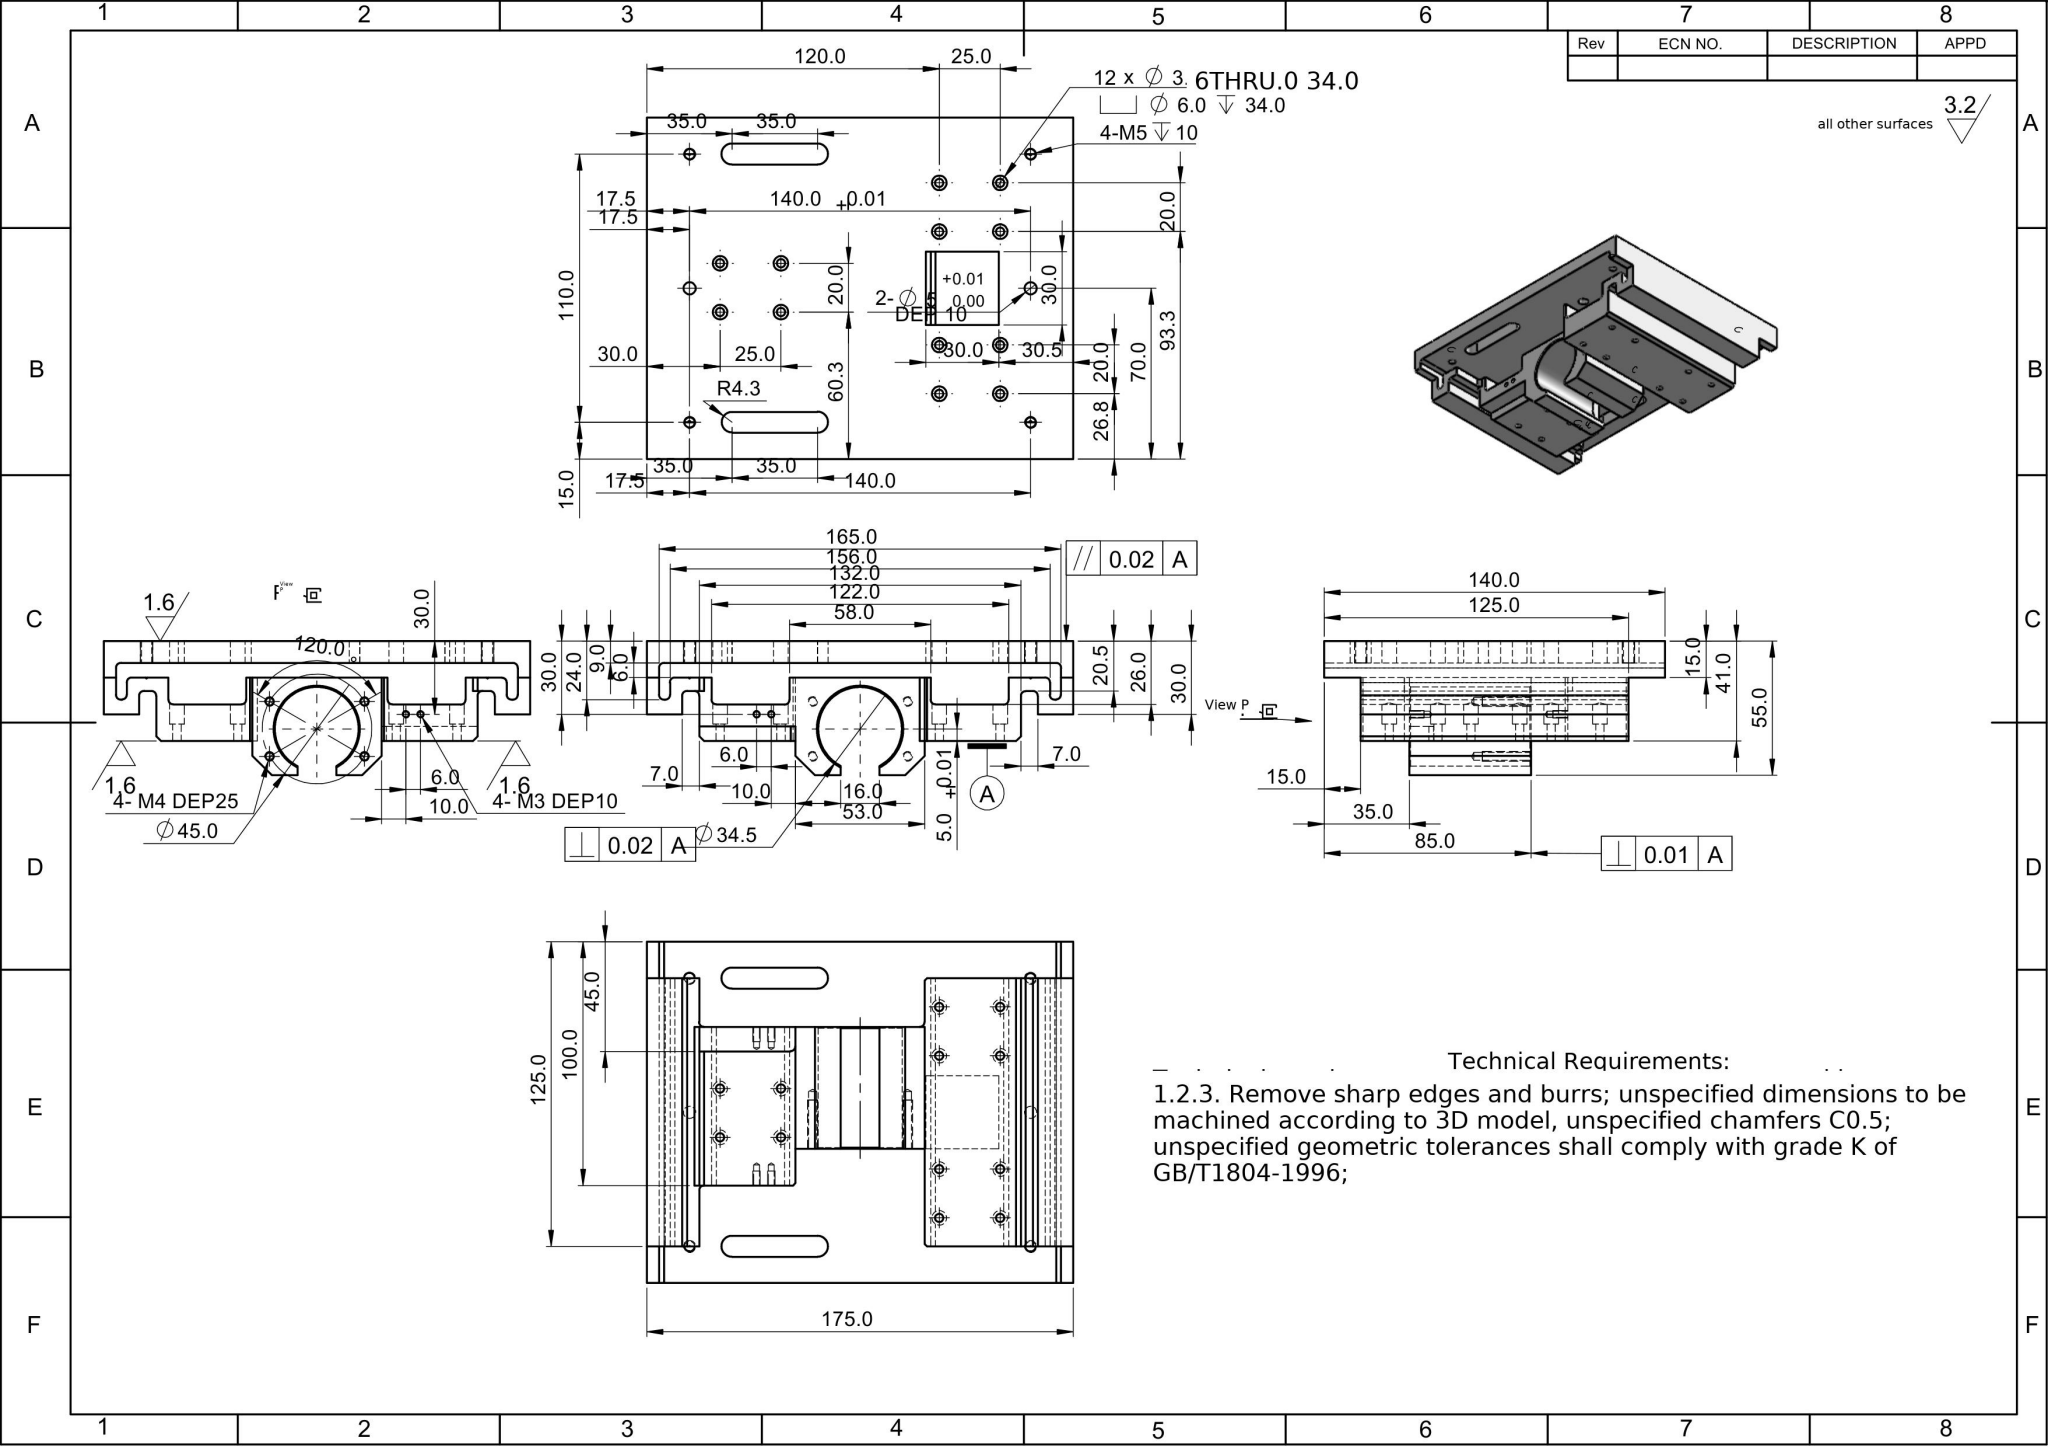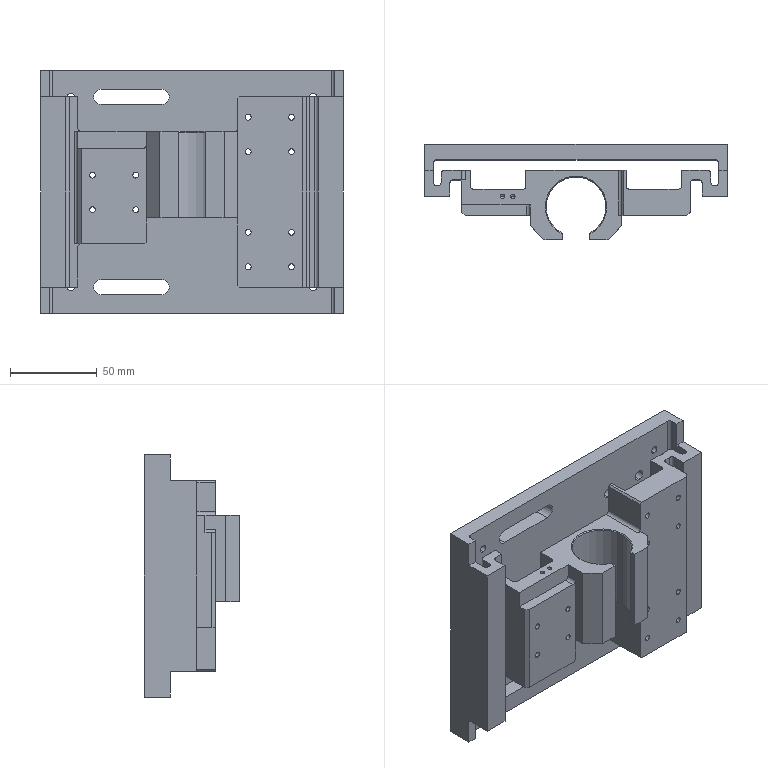Part | SolidWorks | mm | 1 solid | 239 faces | box 175 x 55 x 140 mm | volume 423982 mm3 | cylinder 129 | plane 82 | cone 28 | commonest cylinder face diameters 6 x48 3.4 x24 4 x20 4.2 x8 2.5 x8 3.3 x8 8.6 x6 5 x4
build123d program:
from build123d import *

# Parameters (mm, degrees)
SKETCH1_R                                            = 17.25
BOSS_EXTRUDE1_DEPTH                                  = 70
SKETCH4_W                                            = 39.5
SKETCH4_H                                            = 140
BOSS_EXTRUDE2_DEPTH                                  = 11
SKETCH5_W                                            = 32
SKETCH5_H                                            = 11
CUT_EXTRUDE1_DEPTH                                   = 176.285
SKETCH6_W                                            = 16
SKETCH6_H                                            = 6
CUT_EXTRUDE2_DEPTH                                   = 176.285
SKETCH7_W                                            = 177.5
SKETCH7_H                                            = 40
CUT_EXTRUDE3_DEPTH                                   = 15
SKETCH8_W                                            = 92.5
SKETCH8_H                                            = 20
CUT_EXTRUDE4_DEPTH                                   = 40
FILLET1_R                                            = 2
FILLET2_R                                            = 2
FILLET3_R                                            = 2
CHAMFER1_SIZE                                        = 2
CHAMFER2_SIZE                                        = 1
CHAMFER3_SIZE                                        = 8
CHAMFER4_SIZE                                        = 0.5
HOLE_SIZE_ACCORDING_TO_THE_TYPE_OF_HEXAG_D           = 3.4
HOLE_SIZE_ACCORDING_TO_THE_TYPE_OF_HEXAG_CBORE_D     = 6
HOLE_SIZE_ACCORDING_TO_THE_TYPE_OF_HEXAG_CBORE_DEPTH = 34
M4_TAPPED_HOLE1_D                                    = 3.3
M4_TAPPED_HOLE1_DEPTH                                = 23.5
M4_TAPPED_HOLE1_TIP                                  = 0.9914
M3_TAPPED_HOLE1_D                                    = 2.5
M3_TAPPED_HOLE1_DEPTH                                = 8.5
M3_TAPPED_HOLE1_TIP                                  = 0.7511
M3_TAPPED_HOLE2_D                                    = 2.5
M3_TAPPED_HOLE2_DEPTH                                = 8.5
M3_TAPPED_HOLE2_TIP                                  = 0.7511
SKETCH18_W                                           = 39.5
SKETCH18_H                                           = 6
CUT_EXTRUDE6_DEPTH                                   = 10
CUT_EXTRUDE7_REACH                                   = 122.83
SKETCH19_W                                           = 2.5
SKETCH19_H                                           = 140
FILLET4_R                                            = 2
M5_TAPPED_HOLE1_D                                    = 4.2
M5_TAPPED_HOLE1_DEPTH                                = 14
M5_TAPPED_HOLE1_TIP                                  = 1.262
F_5_0_5_DIAMETER_HOLE1_D                             = 5
F_5_0_5_DIAMETER_HOLE1_DEPTH                         = 10
F_5_0_5_DIAMETER_HOLE1_TIP                           = 1.502
CUT_EXTRUDE8_DEPTH                                   = 10
SKETCH25_W                                           = 30
SKETCH25_H                                           = 30
CUT_EXTRUDE9_DEPTH                                   = 10


with BuildPart() as part:
    # Sketch1 → Boss-Extrude1 (new, symmetric)
    with BuildSketch(Plane.XY):
        Polygon((-90, 0), (90, 0), (90, -15), (87.5, -15), (87.5, -30), (73, -30), (73, -20.5), (66, -20.5), (66, -30), (26.5, -30), (26.5, -55), (-26.5, -55), (-26.5, -30), (-66, -30), (-66, -20.5), (-73, -20.5), (-73, -30), (-87.5, -30), (-87.5, -15), (-90, -15), align=None)
        with Locations((0, -36)):
            Circle(SKETCH1_R, mode=Mode.SUBTRACT)
        Polygon((-82.5, -24), (-82.5, -9), (82.5, -9), (82.5, -24), (78, -24), (78, -15), (-78, -15), (-78, -24), align=None, mode=Mode.SUBTRACT)
    extrude(amount=BOSS_EXTRUDE1_DEPTH, both=True)

    # Sketch4 → Boss-Extrude2 (add)
    with BuildSketch(Plane.XZ.offset(30)):
        with Locations((-46.25, 0)):
            Rectangle(SKETCH4_W, SKETCH4_H)
        with Locations((46.25, 0)):
            Rectangle(SKETCH4_W, SKETCH4_H)
    extrude(amount=BOSS_EXTRUDE2_DEPTH)

    # Sketch5 → Cut-Extrude1 (cut, through all)
    with BuildSketch(Plane.XY.offset(70)):
        with Locations((-45, -20.5)):
            Rectangle(SKETCH5_W, SKETCH5_H)
    cut_extrude1 = extrude(amount=-CUT_EXTRUDE1_DEPTH, mode=Mode.SUBTRACT)

    # Mirror1: Cut-Extrude1 across plane
    add(cut_extrude1.mirror(Plane(origin=(0, 0, 0), x_dir=(0, 0, 1), z_dir=(1, 0, 0))), mode=Mode.SUBTRACT)

    # Sketch6 → Cut-Extrude2 (cut, through all)
    with BuildSketch(Plane(origin=(0, 0, -70), x_dir=(-1, 0, 0), z_dir=(0, 0, -1))):
        with Locations((0, -52)):
            Rectangle(SKETCH6_W, SKETCH6_H)
    extrude(amount=-CUT_EXTRUDE2_DEPTH, mode=Mode.SUBTRACT)

    # Sketch7 → Cut-Extrude3 (cut)
    with BuildSketch(Plane.XY.offset(70)):
        with Locations((1.25, -35)):
            Rectangle(SKETCH7_W, SKETCH7_H)
    cut_extrude3 = extrude(amount=-CUT_EXTRUDE3_DEPTH, mode=Mode.SUBTRACT)

    # Mirror2: Cut-Extrude3 across plane
    add(cut_extrude3.mirror(Plane.XY), mode=Mode.SUBTRACT)

    # Sketch8 → Cut-Extrude4 (cut)
    with BuildSketch(Plane.XZ.offset(55)):
        with Locations((-19.75, 45)):
            Rectangle(SKETCH8_W, SKETCH8_H)
        Polygon((26.5, -55), (-66, -55), (-66, -30), (-26.5, -30), (-26.5, -15), (26.5, -15), align=None)
    extrude(amount=-CUT_EXTRUDE4_DEPTH, mode=Mode.SUBTRACT)

    # Fillet1
    fillet1_edges = [part.edges().sort_by_distance(p)[0] for p in [
        (26.5, -28, 35),
        (-66, -17.75, 35),
        (-66, -17.75, -30),
    ]]
    fillet(fillet1_edges, radius=FILLET1_R)

    # Fillet2
    fillet2_edges = [part.edges().sort_by_distance(p)[0] for p in [
        (-82.5, -24, 0),
        (82.5, -24, 0),
        (78, -24, 0),
        (-78, -24, 0),
        (73, -20.5, 0),
        (66, -20.5, 0),
        (-73, -20.5, 0),
        (29, -26, 0),
        (61, -26, 0),
        (-66, -20.5, 2.5),
        (-61, -26, 2.5),
        (-29, -26, 2.5),
        (82.5, -9, 0),
        (-82.5, -9, 0),
    ]]
    fillet(fillet2_edges, radius=FILLET2_R)

    # Fillet3
    fillet3_edges = [part.edges().sort_by_distance(p)[0] for p in [
        (78, -15, 0),
        (-78, -15, 0),
    ]]
    fillet(fillet3_edges, radius=FILLET3_R)

    # Chamfer1
    chamfer1_edges = [part.edges().sort_by_distance(p)[0] for p in [
        (66, -41, 0),
        (-66, -41, 2.5),
    ]]
    chamfer(chamfer1_edges, length=CHAMFER1_SIZE)

    # Chamfer2
    chamfer2_edges = [part.edges().sort_by_distance(p)[0] for p in [
        (26.5, -28, 55),
        (26.5, -28, -55),
        (-26.5, -28, -30),
    ]]
    chamfer(chamfer2_edges, length=CHAMFER2_SIZE)

    # Chamfer3
    chamfer3_edges = [part.edges().sort_by_distance(p)[0] for p in [
        (26.5, -55, 10),
        (-26.5, -55, 10),
    ]]
    chamfer(chamfer3_edges, length=CHAMFER3_SIZE)

    # Chamfer4
    chamfer4_edges = [part.edges().sort_by_distance(p)[0] for p in [
        (0, -18.75, 35),
        (0, -18.75, -15),
    ]]
    chamfer(chamfer4_edges, length=CHAMFER4_SIZE)

    # Hole Size according to the type of hexag (through all)
    with Locations(Plane(origin=(0, 0, 0), x_dir=(-1, 0, 0), z_dir=(0, 1, 0))):
        with Locations((-32.5, -43.25), (-57.5, -43.25), (-32.5, -23.25), (-57.5, -23.25), (-32.5, 23.25), (-57.5, 23.25), (-32.5, 43.25), (-57.5, 43.25), (57.5, -10.25), (32.5, -10.25), (32.5, 9.75), (57.5, 9.75)):
            CounterBoreHole(HOLE_SIZE_ACCORDING_TO_THE_TYPE_OF_HEXAG_D / 2, HOLE_SIZE_ACCORDING_TO_THE_TYPE_OF_HEXAG_CBORE_D / 2, HOLE_SIZE_ACCORDING_TO_THE_TYPE_OF_HEXAG_CBORE_DEPTH)

    # M4 Tapped Hole1
    with Locations(Plane(origin=(0, 0, -15), x_dir=(-1, 0, 0), z_dir=(0, 0, -1))):
        with Locations((-19.486, -47.25), (19.486, -47.25), (19.486, -24.75), (-19.486, -24.75)):
            Hole(M4_TAPPED_HOLE1_D / 2, depth=M4_TAPPED_HOLE1_DEPTH)
            with Locations((0, 0, -(M4_TAPPED_HOLE1_DEPTH + M4_TAPPED_HOLE1_TIP / 2))):  # 118° drill point
                Cone(0, M4_TAPPED_HOLE1_D / 2, M4_TAPPED_HOLE1_TIP, mode=Mode.SUBTRACT)

    # M3 Tapped Hole1
    with Locations(Plane(origin=(0, 0, -30), x_dir=(-1, 0, 0), z_dir=(0, 0, -1))):
        with Locations((42.5, -30), (36.5, -30)):
            Hole(M3_TAPPED_HOLE1_D / 2, depth=M3_TAPPED_HOLE1_DEPTH)
            with Locations((0, 0, -(M3_TAPPED_HOLE1_DEPTH + M3_TAPPED_HOLE1_TIP / 2))):  # 118° drill point
                Cone(0, M3_TAPPED_HOLE1_D / 2, M3_TAPPED_HOLE1_TIP, mode=Mode.SUBTRACT)

    # M3 Tapped Hole2
    with Locations(Plane.XY.offset(35)):
        with Locations((-42.5, -30), (-36.5, -30)):
            Hole(M3_TAPPED_HOLE2_D / 2, depth=M3_TAPPED_HOLE2_DEPTH)
            with Locations((0, 0, -(M3_TAPPED_HOLE2_DEPTH + M3_TAPPED_HOLE2_TIP / 2))):  # 118° drill point
                Cone(0, M3_TAPPED_HOLE2_D / 2, M3_TAPPED_HOLE2_TIP, mode=Mode.SUBTRACT)

    # Sketch18 → Cut-Extrude6 (cut)
    with BuildSketch(Plane.XY.offset(35)):
        with Locations((-46.25, -38)):
            Rectangle(SKETCH18_W, SKETCH18_H)
    extrude(amount=-CUT_EXTRUDE6_DEPTH, mode=Mode.SUBTRACT)

    # Sketch19 → Cut-Extrude7 (cut, up to next)
    with BuildSketch(Plane.XZ.offset(15), mode=Mode.PRIVATE) as cut_extrude7_sk1:
        with Locations((-88.75, 0)):
            Rectangle(SKETCH19_W, SKETCH19_H)
    cut_extrude7_tool1 = extrude(cut_extrude7_sk1.sketch, amount=-CUT_EXTRUDE7_REACH, mode=Mode.PRIVATE) & part.part
    # Sketch19 → Cut-Extrude7 (cut, up to next)
    with BuildSketch(Plane.XZ.offset(15), mode=Mode.PRIVATE) as cut_extrude7_sk2:
        with Locations((88.75, 0)):
            Rectangle(SKETCH19_W, SKETCH19_H)
    cut_extrude7_tool2 = extrude(cut_extrude7_sk2.sketch, amount=-CUT_EXTRUDE7_REACH, mode=Mode.PRIVATE) & part.part
    add(cut_extrude7_tool1.solids().sort_by_distance((-88.75, -15, 0))[0], mode=Mode.SUBTRACT)
    add(cut_extrude7_tool2.solids().sort_by_distance((88.75, -15, 0))[0], mode=Mode.SUBTRACT)

    # Fillet4
    fillet4_edges = [part.edges().sort_by_distance(p)[0] for p in [
        (-26.5, -38, 25),
    ]]
    fillet(fillet4_edges, radius=FILLET4_R)

    # M5 Tapped Hole1
    with Locations(Plane(origin=(0, 0, 0), x_dir=(-1, 0, 0), z_dir=(0, 1, 0))):
        with Locations((-70, -55), (-70, 55), (70, 55), (70, -55)):
            Hole(M5_TAPPED_HOLE1_D / 2, depth=M5_TAPPED_HOLE1_DEPTH)
            with Locations((0, 0, -(M5_TAPPED_HOLE1_DEPTH + M5_TAPPED_HOLE1_TIP / 2))):  # 118° drill point
                Cone(0, M5_TAPPED_HOLE1_D / 2, M5_TAPPED_HOLE1_TIP, mode=Mode.SUBTRACT)

    # 5.0 _5_ Diameter Hole1
    with Locations(Plane(origin=(0, 0, 0), x_dir=(-1, 0, 0), z_dir=(0, 1, 0))):
        with Locations((70, 0), (-70, 0)):
            Hole(F_5_0_5_DIAMETER_HOLE1_D / 2, depth=F_5_0_5_DIAMETER_HOLE1_DEPTH)
            with Locations((0, 0, -(F_5_0_5_DIAMETER_HOLE1_DEPTH + F_5_0_5_DIAMETER_HOLE1_TIP / 2))):  # 118° drill point
                Cone(0, F_5_0_5_DIAMETER_HOLE1_D / 2, F_5_0_5_DIAMETER_HOLE1_TIP, mode=Mode.SUBTRACT)

    # Sketch24 → Cut-Extrude8 (cut)
    with BuildSketch(Plane(origin=(0, 0, 0), x_dir=(1, 0, 0), z_dir=(0, 1, 0))):
        with BuildLine():
            Line((-52.5, -50.7), (-17.5, -50.7))
            ThreePointArc((-17.5, -50.7), (-13.2, -55), (-17.5, -59.3))
            Line((-17.5, -59.3), (-52.5, -59.3))
            ThreePointArc((-52.5, -59.3), (-56.8, -55), (-52.5, -50.7))
        make_face()
        with BuildLine():
            Line((-52.5, 59.3), (-17.5, 59.3))
            ThreePointArc((-17.5, 59.3), (-13.2, 55), (-17.5, 50.7))
            Line((-17.5, 50.7), (-52.5, 50.7))
            ThreePointArc((-52.5, 50.7), (-56.8, 55), (-52.5, 59.3))
        make_face()
    extrude(amount=-CUT_EXTRUDE8_DEPTH, mode=Mode.SUBTRACT)

    # Sketch25 → Cut-Extrude9 (cut)
    with BuildSketch(Plane(origin=(0, 0, 0), x_dir=(1, 0, 0), z_dir=(0, 1, 0))):
        with Locations((42, 0)):
            Rectangle(SKETCH25_W, SKETCH25_H)
    extrude(amount=-CUT_EXTRUDE9_DEPTH, mode=Mode.SUBTRACT)


solid = part.part